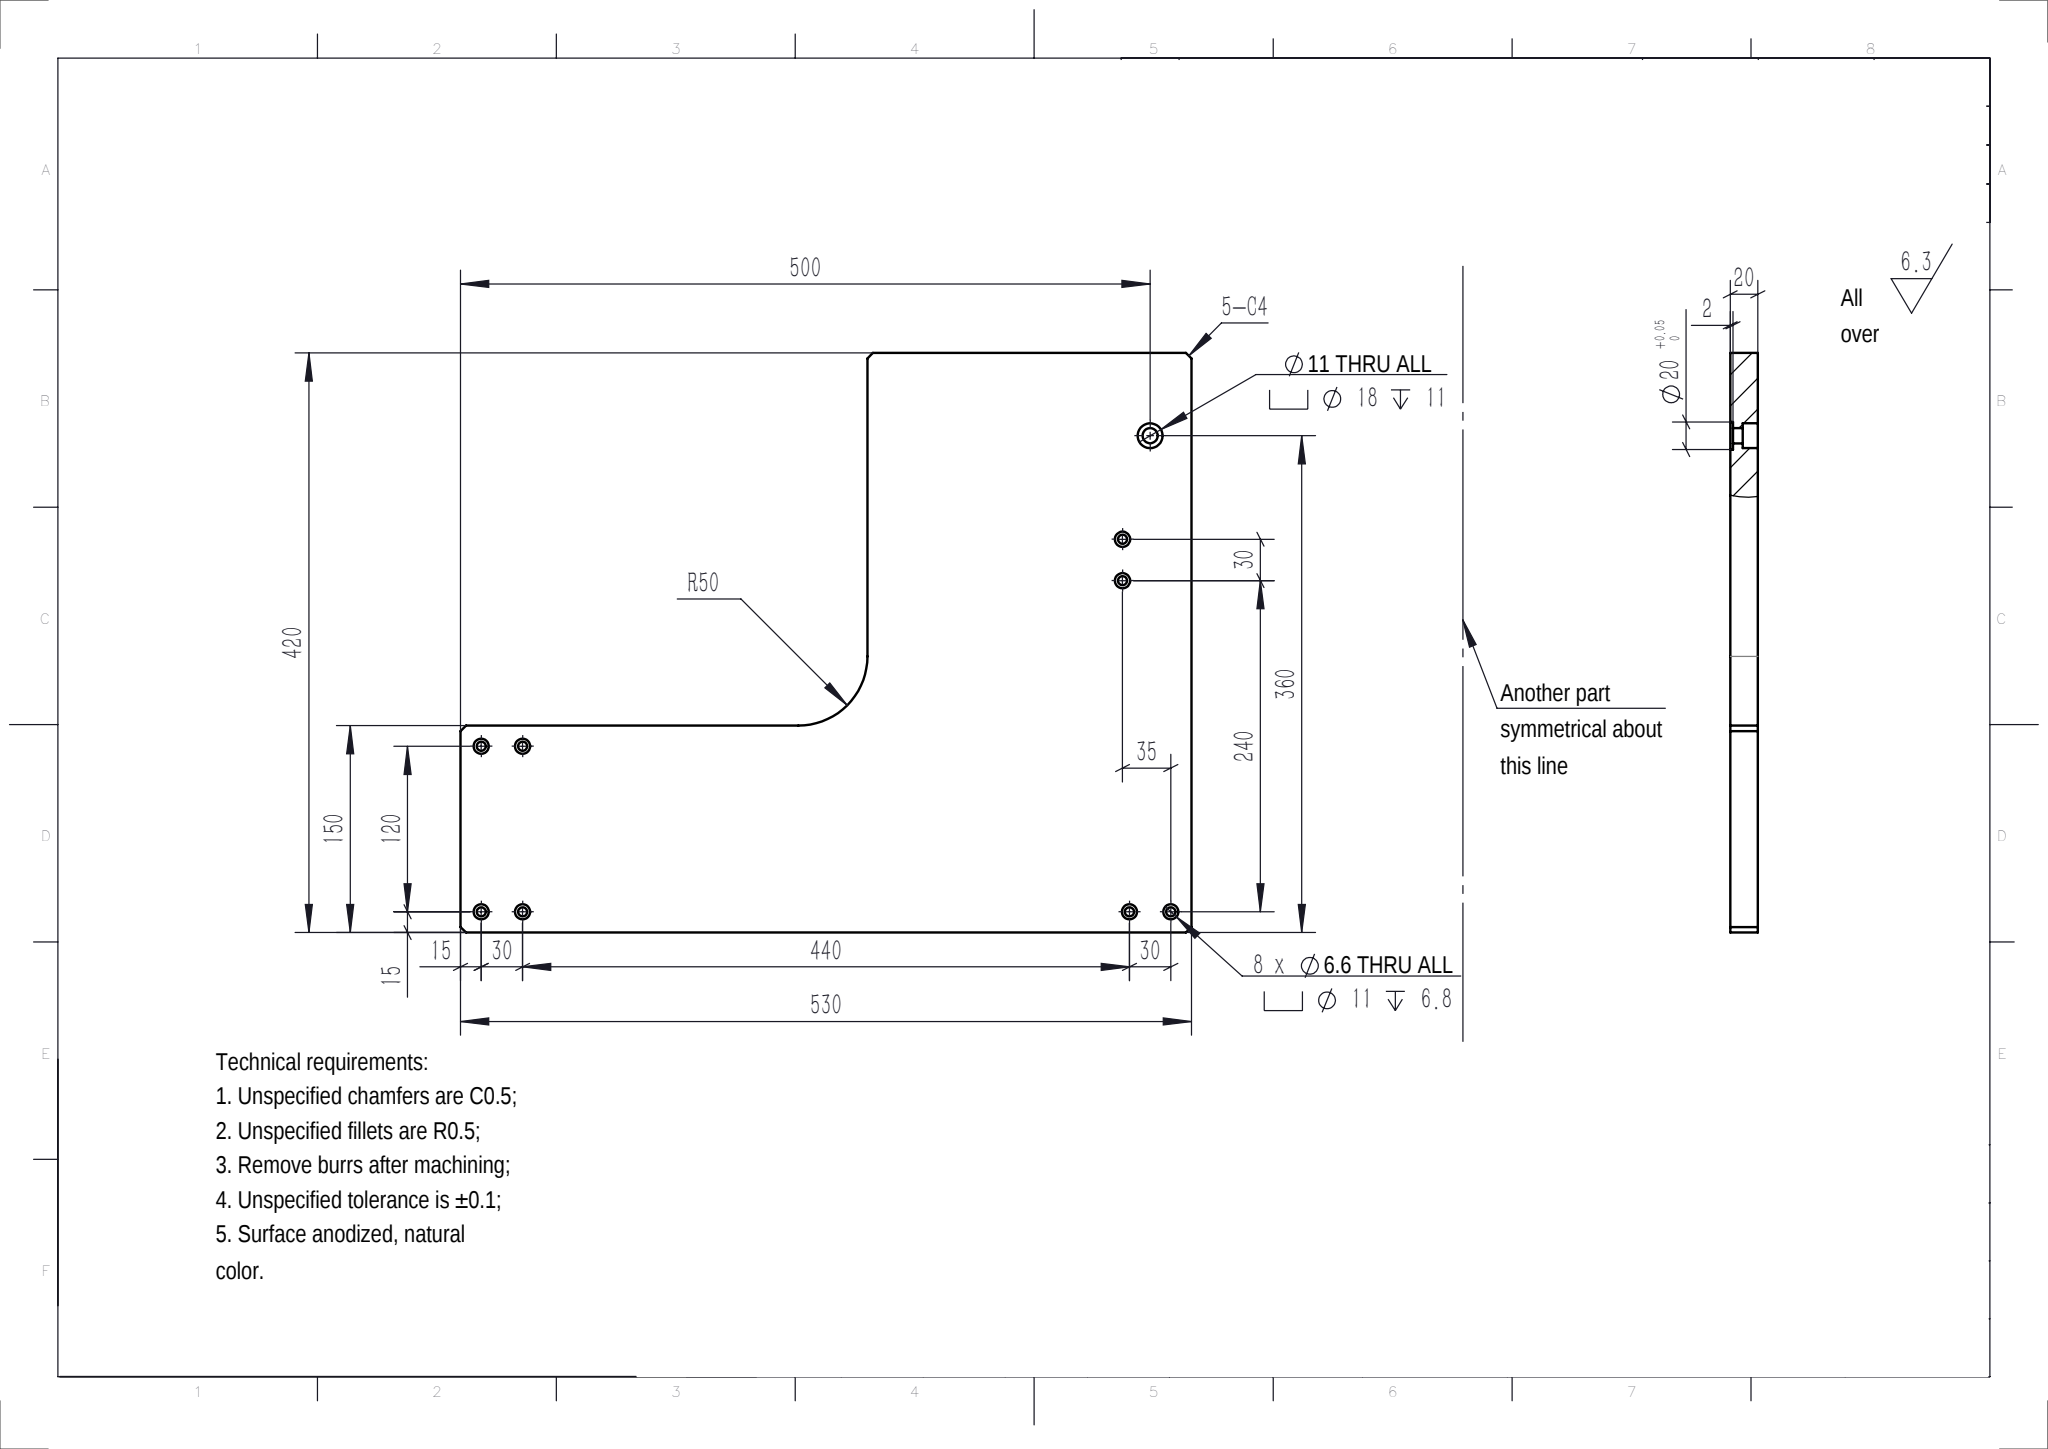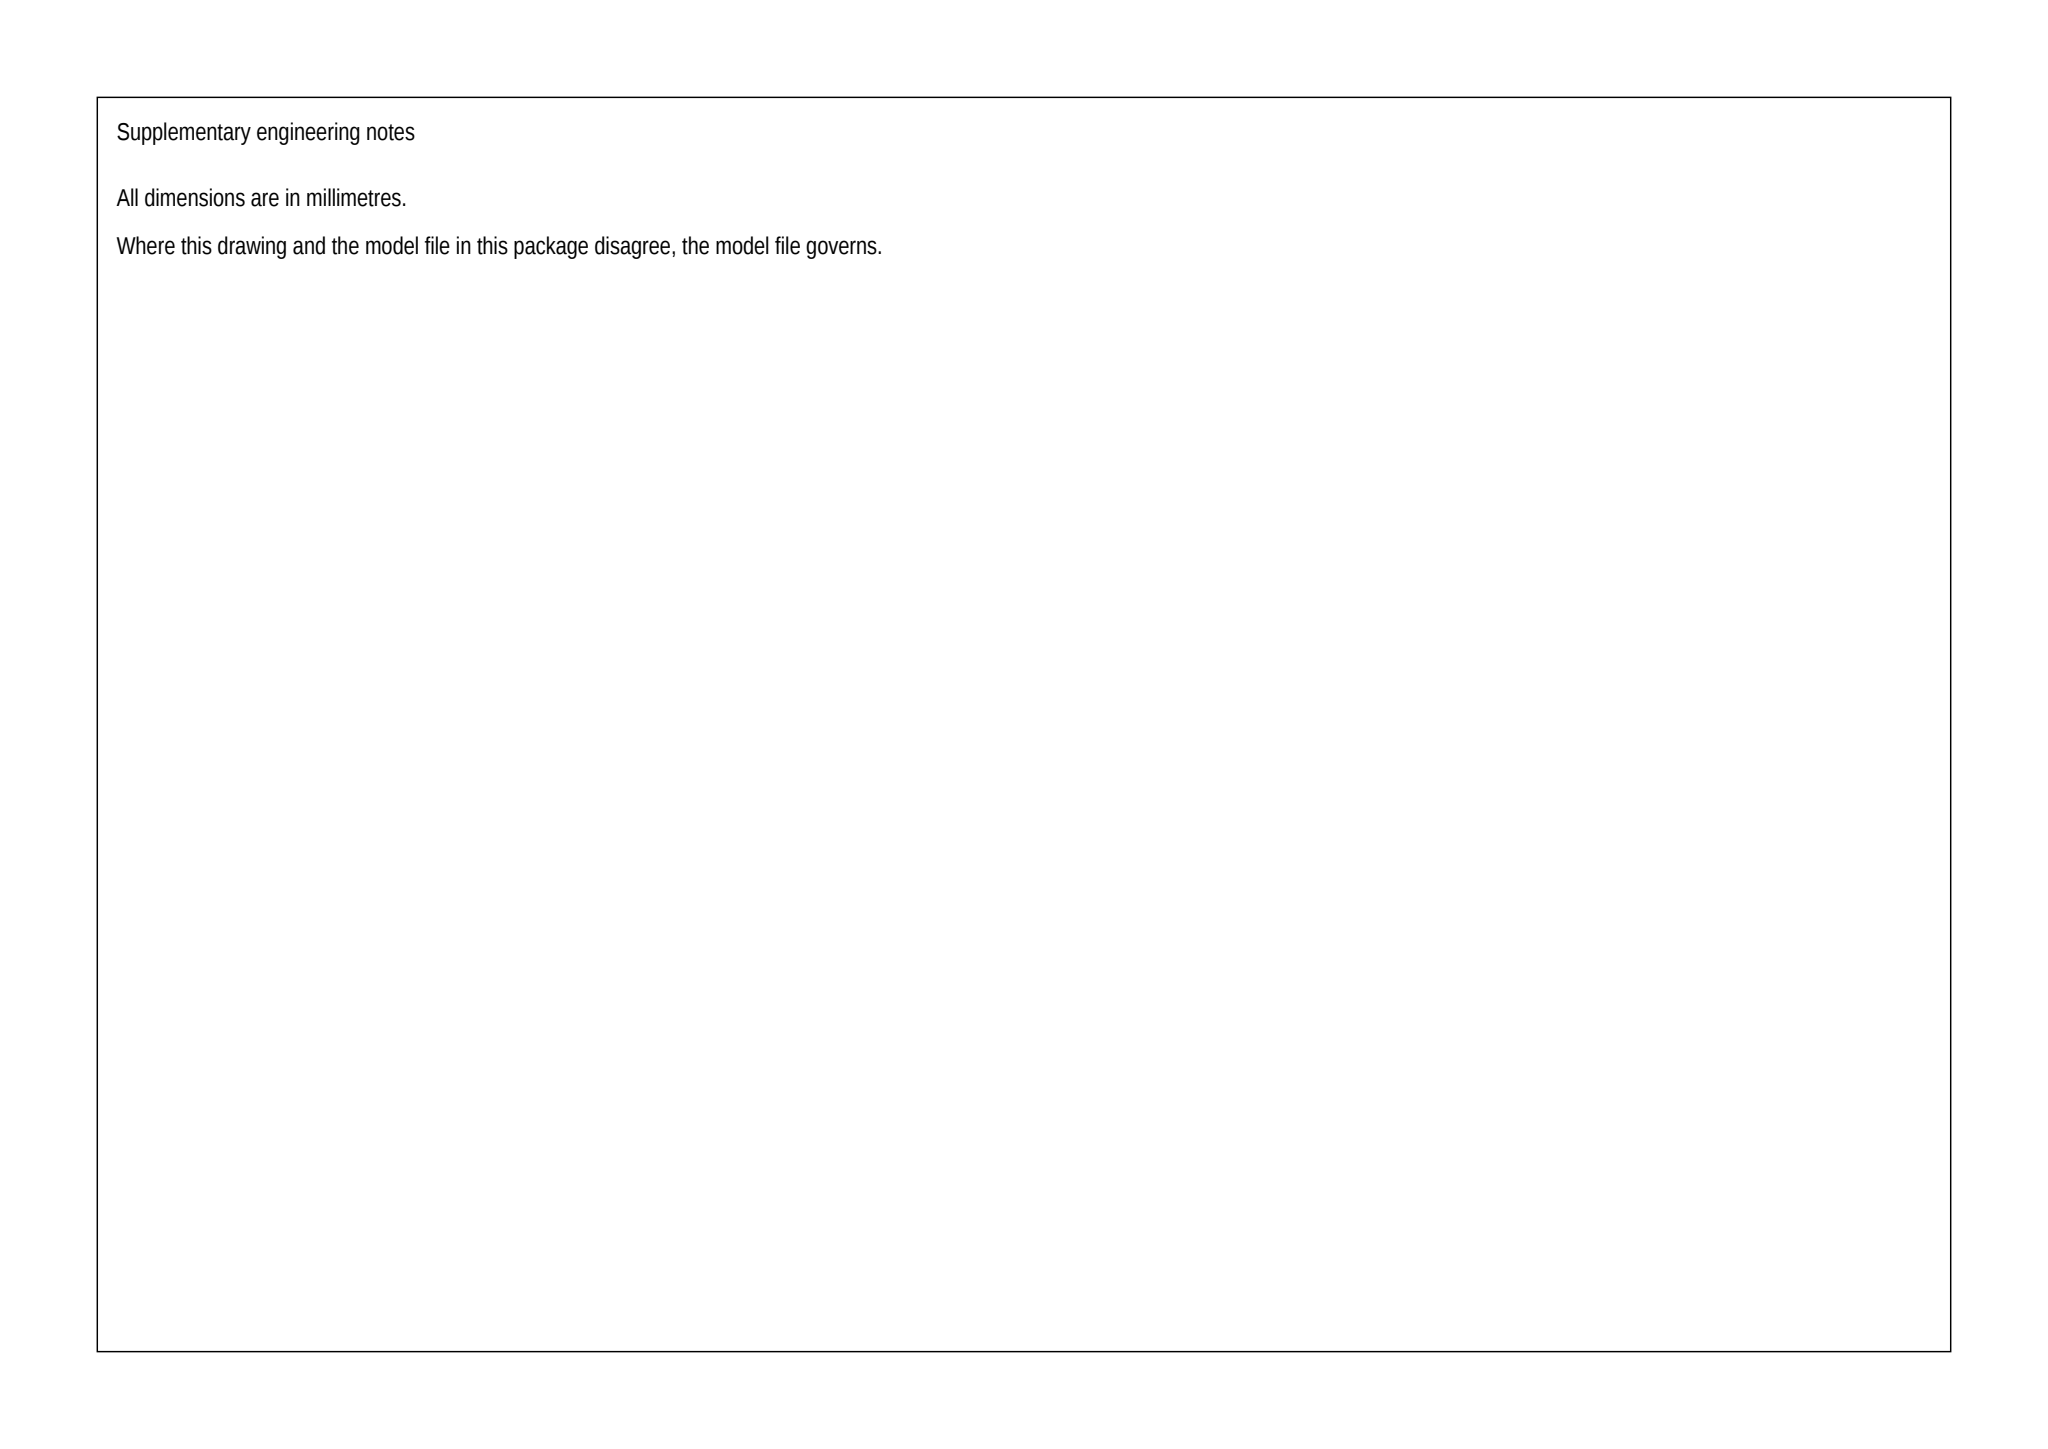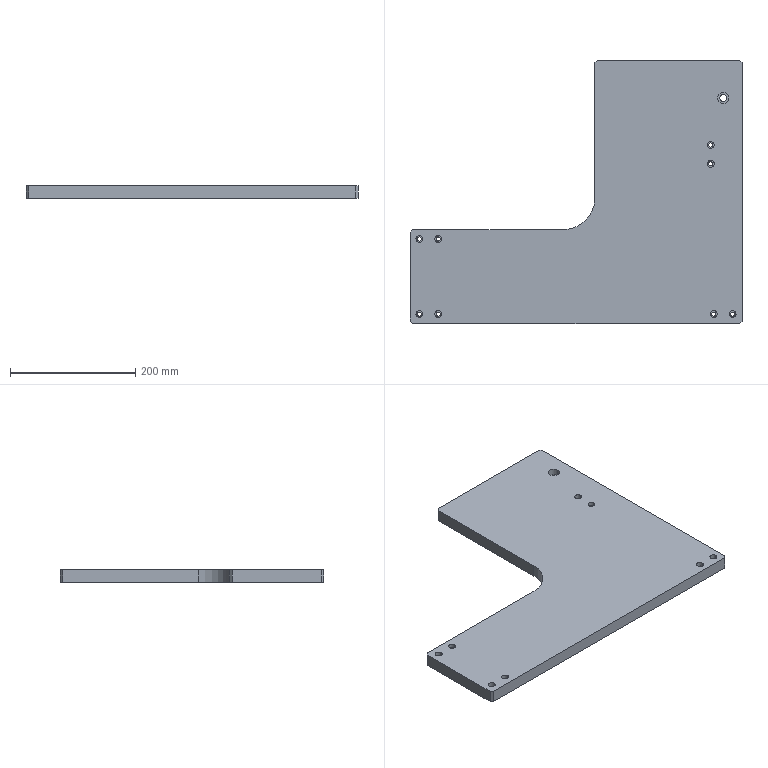Part | SolidWorks | mm | 1 solid | 62 faces | box 530 x 420 x 20 mm | volume 2856055 mm3 | cylinder 39 | plane 23 | commonest cylinder face diameters 11 x18 6.6 x16 20 x2 18 x2 100 x1
build123d program:
from build123d import *

# Parameters (mm, degrees)
BOSS_EXTRUDE1_DEPTH                               = 20
HOLE_SIZE_ACCORDING_TO_HEXAGON_SOCKET_D           = 11
HOLE_SIZE_ACCORDING_TO_HEXAGON_SOCKET_CBORE_D     = 18
HOLE_SIZE_ACCORDING_TO_HEXAGON_SOCKET_CBORE_DEPTH = 11
SKETCH6_R                                         = 10
CUT_EXTRUDE3_DEPTH                                = 2
HOLE_SIZE_ACCORDING_TO_HEXAGON_SO_2_D             = 6.6
HOLE_SIZE_ACCORDING_TO_HEXAGON_SO_2_CBORE_D       = 11
HOLE_SIZE_ACCORDING_TO_HEXAGON_SO_2_CBORE_DEPTH   = 6.8
CHAMFER1_SIZE                                     = 4


with BuildPart() as part:
    # Sketch1 → Boss-Extrude1 (new body)
    with BuildSketch(Plane.XY):
        with BuildLine():
            Line((530, 0), (0, 0))
            Line((0, 0), (0, 150))
            Line((0, 150), (245, 150))
            ThreePointArc((245, 150), (280.355, 164.645), (295, 200))
            Line((295, 200), (295, 420))
            Line((295, 420), (530, 420))
            Line((530, 420), (530, 0))
        make_face()
    extrude(amount=BOSS_EXTRUDE1_DEPTH)

    # Hole Size _ according to_ Hexagon Socket (through all)
    with Locations(Plane.XY.offset(20)):
        with Locations((500, 360)):
            CounterBoreHole(HOLE_SIZE_ACCORDING_TO_HEXAGON_SOCKET_D / 2, HOLE_SIZE_ACCORDING_TO_HEXAGON_SOCKET_CBORE_D / 2, HOLE_SIZE_ACCORDING_TO_HEXAGON_SOCKET_CBORE_DEPTH)

    # Sketch6 → Cut-Extrude3 (cut)
    with BuildSketch(Plane(origin=(0, 0, 0), x_dir=(-1, 0, 0), z_dir=(0, 0, -1))):
        with Locations((-500, 360)):
            Circle(SKETCH6_R)
    extrude(amount=-CUT_EXTRUDE3_DEPTH, mode=Mode.SUBTRACT)

    # Hole Size _ according to_ Hexagon So 2 (through all)
    with Locations(Plane.XY.offset(20)):
        with Locations((480, 285), (480, 255), (15, 15), (45, 15), (485, 15), (515, 15), (15, 135), (45, 135)):
            CounterBoreHole(HOLE_SIZE_ACCORDING_TO_HEXAGON_SO_2_D / 2, HOLE_SIZE_ACCORDING_TO_HEXAGON_SO_2_CBORE_D / 2, HOLE_SIZE_ACCORDING_TO_HEXAGON_SO_2_CBORE_DEPTH)

    # Chamfer1
    chamfer1_edges = [part.edges().sort_by_distance(p)[0] for p in [
        (0, 150, 10),
        (295, 420, 10),
        (530, 420, 10),
        (530, 0, 10),
        (0, 0, 10),
    ]]
    chamfer(chamfer1_edges, length=CHAMFER1_SIZE)


solid = part.part